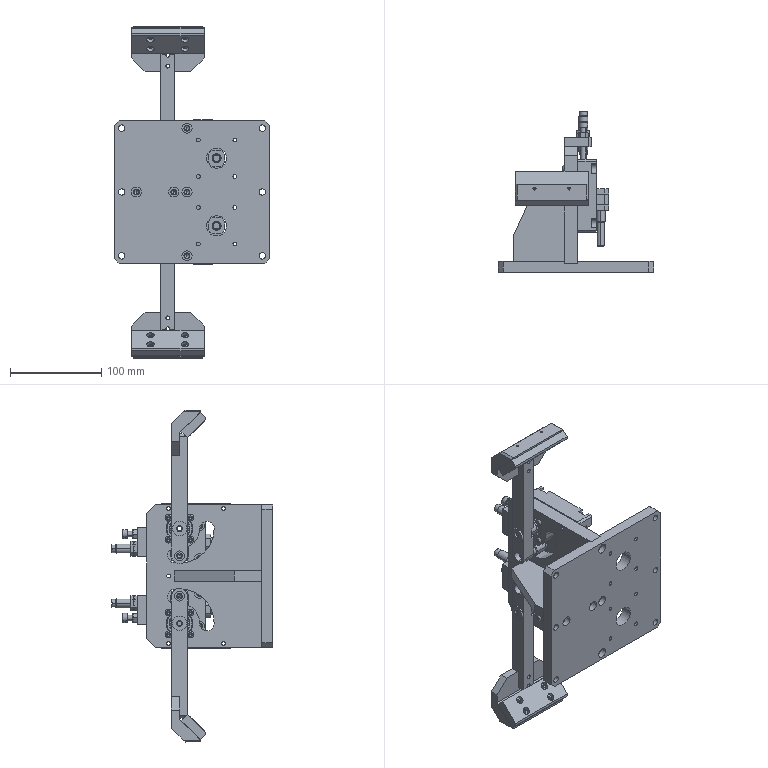Assembly | SolidWorks | mm | 57 component files | 57 solids | 1432 faces | box 170 x 176.7 x 364.01 mm | volume 992692 mm3 | plane 567 | cylinder 496 | spline 179 | cone 174 | torus 16 | commonest cylinder face diameters 10 x64 4.2 x48 4 x32 5 x28 5.5 x28 11 x26 16 x22 6.6 x22
Bill of materials:
A26 | 2 | S45C | Plate of constant thickness bent once into two flat legs at an obtuse angle. The shorter leg has angled (chamfered) corners and two round holes; the longer rectangular leg has four smaller holes in a 2x2 pattern.
A27 | 2 | Urethane | Rectangular flat bar or plate with four counterbored holes in a 2x2 pattern; one end face appears to be cut at an angle.
A73 | 4 | S45C | Thin flat ring (annular disc) with a centered round through hole, like a plain washer.
A74 | 2 | S45C | Stepped round pin with three coaxial diameters: a large head with a chamfered end, a middle shank, and a smaller end shank with a small axial hole.
A75 | 2 | Brass | Plain cylindrical sleeve or bushing with a large through bore and chamfered outer edges at both ends.
A78 | 2 | S45C | Thin flat ring (annular disc) with a centered round through hole, like a plain washer; the hole is a little smaller relative to the outside diameter than in the similar ring.
A79 | 2 | S45C | Thicker flat ring or spacer disc with a fairly small centered through hole.
A87 | 1 | S45C | Long flat bar or link with one rounded end. It has a hole near the rounded end, a larger hole partway along, a stepped or notched side profile, and a narrower tail section with two small holes and a chamfered tip.
BPS01-d6 | 2 | Standard Part | Short thick cylinder or roller-like ring with a centered through bore, rounded or chamfered outer edges, and a small edge break at the bore.
A70 | 1 | S136 | Thick rectangular plate with two clipped corners on one side. It has two mirrored curved arc slots, two large round holes, a row of small and medium holes across the middle, small holes near the edges, and holes drilled into one edge face.
A72 | 2 | S45C | Stepped cylindrical bushing with a through bore. It has a large central collar with a small extra step on one side, and two shaft ends of different diameters with chamfered ends.
A76 | 2 | S136 | Rectangular block or plate with two clipped corners on one side, a large obround (stadium-shaped) through slot, and two round holes in a stepped flange strip along the opposite side.
A77 | 2 | S45C | Thick, nearly square block or plate with two chamfered corners on one side and four through holes: three smaller holes and one larger hole.
A80 | 2 | S45C | Rectangular block with chamfered corners on one long side and a U-shaped slot with a rounded end cut through its full thickness, open on that side.
A81 | 2 | S45C | Stepped shaft or pin on one axis, with two spaced flanges that have chamfered corners, a middle shoulder diameter, and a long, smaller-diameter pin end.
A82 | 1 | S45C | Thin rectangular plate with small corner chamfers and a pattern of holes: two large through holes, several medium holes along the edges and center line, and small holes arranged in rows. A shallow notch is cut into one long edge.
A83 | 1 | A6061 | Flat block with a tapered planform: one end is narrowed by an angled cut. Drilled holes enter the long side faces.
A84 | 2 | S136 | Long rectangular bar with a raised step or tab region at one end of the profile, rounded-end notches cut into one side face, and two through holes along its length. The end corners are chamfered.
A85 | 1 | S136 | Long rectangular bar similar to a spacer or clamp bar, with two through holes near the ends, chamfered end corners, and a small stepped notch along one edge.
DeepGrooveBallBearing16001 | 2 | Standard Part | Annular rolling-element assembly: an outer ring, an inner ring and a single row of spherical balls between them. No cage or seals are visible. The geometry is consistent with a radial ball bearing.
M5X10 | 1 | Standard Part | Fastener-like part with a domed (button) head, a hexagonal socket recess and a plain cylindrical shank.
M6-N | 2 | Standard Part | Hexagonal nut-like part with a round central bore and chamfered corners on both faces.
M6X35-N | 2 | Standard Part | Headed cylindrical pin or simplified screw: a short cylindrical head of larger diameter with a long, plain, smaller-diameter shank.
PanHeadM4X8-N | 8 | Standard Part | Round-head, rivet- or pin-like part: a domed head with a flat underside and a plain cylindrical shank with a flat end.
RB1006-1 | 2 |  | Elongated, stepped cylindrical body. A long main barrel sits between a short, slightly narrower end section on one side and a short stepped collar on the other. A small solid cylindrical pin sticks out along the axis from the collar end. The opposite end section has a small notch or slot cut into its edge.
RB1006-2 | 2 |  | Thin hexagonal ring with a large plain central through-bore. The outer corners are chamfered on both faces, which leaves curved boundaries on the side flats. Its overall shape matches a thin hex nut.
RB1006-3 | 2 |  | Thin hexagonal ring with a large plain central through-bore. The outer corners are chamfered on both faces, which leaves curved boundaries on the side flats. Its overall shape matches a thin hex nut.
A89 | 1 | S45C | Long, narrow bar or plate with a roughly rectangular cross-section. One end is chamfered and squared off, and the other end is fully rounded. There are two small holes near the chamfered end and a larger hole partway down the bar. A side notch or pocket cuts in near the larger hole, and the rounded end has one more hole with an edge recess or counterbore. The bar steps in width near the chamfered end.
Mates:
1. coincident | ClampingAssembly-1/A72-1 face at (-35.551, 66.036, -52.5) dir (-1, 0, 0) | ClampingArm2-1/A87-1 face at (-35.551, 66.025, -85.5) dir (1, 0, 0)
2. parallel | ClampingAssembly-1/A72-1 face at (-37.551, 60.742, -58.498) dir (0, -0.0003333, -1) | ClampingArm2-1/A87-1 face at (-38.051, 75.034, -58.503) dir (0, 0.0003333, 1)
3. concentric | ClampingAssembly-1/A72-1 face at (-49.551, 66.036, -52.5) dir (1, 0, 0) r 5 | ClampingArm2-1/A87-1 face at (-50.551, 66.036, -52.5) dir (1, 0, 0) r 5
4. cam | ClampingAssembly-1/A76-1 face at (-14.551, 56.526, -21.5) dir (0, 1, 0) | ClampingArm2-1/BPS01-d6-1 face at (-2.651, 66.046, -22.5) dir (-1, 0, 0) r 9.5
5. coincident | ClampingArm2-1/A87-1 face at (-50.551, 66.025, -85.5) dir (-1, 0, 0) | Reverse-ClampingArm2-1/A89-1 face at (-50.551, 66.047, 84.5) dir (-1, 0, 0)
6. parallel | ClampingAssembly-1/A72-2 face at (-37.551, 71.329, 57.498) dir (0, 0.0003333, 1) | Reverse-ClampingArm2-1/A89-1 face at (-38.051, 57.038, 57.503) dir (0, -0.0003333, -1)
7. cam | ClampingAssembly-1/A76-3 face at (-14.551, 66.036, 20.5) dir (1, 0, 0) r 9.51 | Reverse-ClampingArm2-1/BPS01-d6-1 face at (-2.651, 66.026, 21.5) dir (-1, 0, 0) r 9.5
8. parallel | ClampingAssembly-1/A72-2 face at (-37.551, 60.742, 45.502) dir (0, -0.0003333, -1) | Reverse-ClampingArm2-1/A89-1 face at (-38.051, 57.034, 45.503) dir (0, 0.0003333, 1)
9. concentric | ClampingAssembly-1/A72-2 face at (-49.551, 66.036, 51.5) dir (1, 0, 0) r 5 | Reverse-ClampingArm2-1/A89-1 face at (-50.551, 66.036, 51.5) dir (1, 0, 0) r 5
10. coincident | A87-1 face at (-0.2508, 28.779, -71) dir (0, 1, 0) | A26-1 face at (47.249, 28.779, -47) dir (0, -1, 0)
11. concentric | A87-1 face at (7.249, 28.779, -53) dir (0, 1, 0) r 2.1 | A26-1 face at (7.249, 37.779, -53) dir (0, 1, 0) r 2.75
12. concentric | A87-1 face at (7.249, 28.779, -65) dir (0, 1, 0) r 2.1 | A26-1 face at (7.249, 37.779, -65) dir (0, 1, 0) r 2.75
13. coincident | A26-1 face at (47.249, 28.779, -72) dir (0, -0.7071, 0.7071) | A27-1 face at (7.249, 16.672, -84.107) dir (0, 0.7071, -0.7071)
14. concentric | A26-1 face at (-11.751, 21.622, -79.157) dir (0, -0.7071, 0.7071) r 1.65 | A27-1 face at (-11.751, 14.551, -72.086) dir (0, -0.7071, 0.7071) r 2.25
15. concentric | A26-1 face at (26.249, 21.622, -79.157) dir (0, -0.7071, 0.7071) r 1.65 | A27-1 face at (26.249, 14.551, -72.086) dir (0, -0.7071, 0.7071) r 2.25
16. coincident | A87-1 face at (-0.2508, 28.779, 0) dir (-1, 0, 0) | A73-1 face at (-0.2508, 28.779, 33) dir (1, 0, 0)
17. concentric | A87-1 face at (-0.2508, 28.779, 33) dir (1, 0, 0) r 5 | A73-1 face at (-0.2508, 28.779, 33) dir (-1, 0, 0) r 3.25
18. concentric | A87-1 face at (-0.2508, 28.779, 63) dir (1, 0, 0) r 3.25 | A74-1 face at (20.749, 28.779, 63) dir (-1, 0, 0) r 7
19. coincident | A87-1 face at (12.749, 28.779, 63) dir (1, 0, 0) | A74-1 face at (12.749, 28.779, 63) dir (-1, 0, 0)
20. concentric | A74-1 face at (35.749, 28.779, 63) dir (-1, 0, 0) r 5 | A75-1 face at (35.249, 28.779, 63) dir (-1, 0, 0) r 8
21. width | A75-1 face at (21.249, 28.779, 63) dir (-1, 0, 0) | A75-1 face at (35.249, 28.779, 63) dir (1, 0, 0) | A74-1 face at (20.749, 28.779, 63) dir (1, 0, 0) | A74-1 face at (35.749, 28.779, 63) dir (1, 0, 0)
22. concentric | A74-1 face at (47.749, 28.779, 63) dir (-1, 0, 0) r 3 | A78-1 face at (37.749, 28.779, 63) dir (-1, 0, 0) r 3.1
23. coincident | A74-1 face at (35.749, 28.779, 63) dir (1, 0, 0) | A78-1 face at (35.749, 28.779, 63) dir (-1, 0, 0)
24. concentric | A74-1 face at (47.749, 28.779, 63) dir (-1, 0, 0) r 3 | BPS01-d6-1 face at (47.649, 28.779, 63) dir (-1, 0, 0) r 9.5
25. coincident | A78-1 face at (37.749, 28.779, 63) dir (1, 0, 0) | BPS01-d6-1 face at (37.749, 28.779, 63) dir (-1, 0, 0)
26. coincident | A74-1 face at (47.749, 28.779, 63) dir (1, 0, 0) | A79-1 face at (47.749, 28.779, 63) dir (-1, 0, 0)
27. concentric | A74-1 face at (47.749, 28.779, 63) dir (1, 0, 0) r 1.25 | A79-1 face at (49.749, 28.779, 63) dir (-1, 0, 0) r 5
28. parallel | A87-1 face at (14.749, 37.779, 71) dir (0, 1, 0) | A73-1 plane at (-1.251, 28.779, 33) dir (0, 1, 0)
29. parallel | A87-1 face at (14.749, 37.779, 71) dir (0, 1, 0) | A74-1 plane at (16.749, 28.779, 63) dir (0, -1, 0)
30. parallel | A87-1 face at (14.749, 37.779, 71) dir (0, 1, 0) | A75-1 plane at (28.249, 28.779, 63) dir (0, -1, 0)
31. parallel | A87-1 face at (14.749, 37.779, 71) dir (0, 1, 0) | A78-1 plane at (35.749, 28.779, 63) dir (0, 1, 0)
32. parallel | A87-1 face at (14.749, 37.779, 71) dir (0, 1, 0) | BPS01-d6-1 plane at (42.749, 28.779, 63) dir (0, -1, 0)
33. parallel | A87-1 face at (14.749, 37.779, 71) dir (0, 1, 0) | A79-1 plane at (48.749, 28.779, 63) dir (0, 1, 0)
34. concentric | A70-1 face at (7.478, 54.35, -52) dir (-1, 0, 0) r 14 | DeepGrooveBallBearing16001-1 face at (-4.733, 54.35, -52) dir (-1, 0, 0) r 14
35. coincident | A70-1 face at (7.478, 54.35, -52) dir (-1, 0, 0) | DeepGrooveBallBearing16001-1 face at (7.478, 68.35, -52) dir (1, 0, 0)
36. parallel | A70-1 face at (15.478, 90.35, -78) dir (0, 0, -1) | DeepGrooveBallBearing16001-1 plane at (3.978, 54.35, -52) dir (0, 0, 1)
37. concentric | DeepGrooveBallBearing16001-1 face at (-2.994, 54.35, -52) dir (-1, 0, 0) r 6 | A72-1 face at (7.478, 54.35, -52) dir (-1, 0, 0) r 6
38. coincident | DeepGrooveBallBearing16001-1 face at (0.4778, 63.017, -52) dir (-1, 0, 0) | A72-1 face at (0.4778, 54.35, -52) dir (1, 0, 0)
39. concentric | A70-1 face at (0.4778, 66.371, -64.021) dir (-1, 0, 0) r 2 | PanHeadM4X8-N-1 face at (8.478, 66.371, -64.021) dir (-1, 0, 0) r 2
40. coincident | A70-1 face at (0.4778, 26.35, 0) dir (-1, 0, 0) | PanHeadM4X8-N-1 face at (0.4778, 66.371, -64.021) dir (1, 0, 0)
41. parallel | A70-1 face at (15.478, 90.35, -78) dir (0, 0, -1) | PanHeadM4X8-N-1 face at (-0.4222, 67.093, -62.771) dir (0, 0, -1)
42. concentric | A70-1 face at (0.4778, 42.329, -64.021) dir (-1, 0, 0) r 2 | PanHeadM4X8-N-2 face at (8.478, 42.329, -64.021) dir (-1, 0, 0) r 2
43. coincident | A70-1 face at (0.4778, 26.35, 0) dir (-1, 0, 0) | PanHeadM4X8-N-2 face at (0.4778, 42.329, -64.021) dir (1, 0, 0)
44. parallel | A70-1 face at (15.478, 90.35, -78) dir (0, 0, -1) | PanHeadM4X8-N-2 face at (-0.4222, 43.051, -62.771) dir (0, 0, -1)
45. concentric | A70-1 face at (0.4778, 42.329, -39.979) dir (-1, 0, 0) r 2 | PanHeadM4X8-N-4 face at (8.478, 42.329, -39.979) dir (-1, 0, 0) r 2
46. coincident | A70-1 face at (0.4778, 26.35, 0) dir (-1, 0, 0) | PanHeadM4X8-N-4 face at (0.4778, 42.329, -39.979) dir (1, 0, 0)
47. parallel | A70-1 face at (15.478, 90.35, -78) dir (0, 0, -1) | PanHeadM4X8-N-4 face at (-0.4222, 43.051, -38.729) dir (0, 0, -1)
48. concentric | A70-1 face at (0.4778, 66.371, -39.979) dir (-1, 0, 0) r 2 | PanHeadM4X8-N-6 face at (8.478, 66.371, -39.979) dir (-1, 0, 0) r 2
49. coincident | A70-1 face at (0.4778, 26.35, 0) dir (-1, 0, 0) | PanHeadM4X8-N-6 face at (0.4778, 66.371, -39.979) dir (1, 0, 0)
50. parallel | A70-1 face at (15.478, 90.35, -78) dir (0, 0, -1) | PanHeadM4X8-N-6 face at (-0.4222, 67.093, -38.729) dir (0, 0, -1)
51. coincident | A72-1 face at (7.478, 54.35, -52) dir (1, 0, 0) | A73-1 face at (7.478, 54.35, -52) dir (-1, 0, 0)
52. concentric | A72-1 face at (7.478, 54.35, -52) dir (1, 0, 0) r 2.5 | A73-1 face at (9.478, 54.35, -52) dir (-1, 0, 0) r 3.25
53. coincident | A70-1 face at (15.478, 26.35, 0) dir (1, 0, 0) | A76-1 face at (15.478, 51.35, -37) dir (-1, 0, 0)
54. coincident | A73-1 face at (9.478, 54.35, -52) dir (1, 0, 0) | M5X10-1 face at (9.478, 54.35, -52) dir (-1, 0, 0)
55. concentric | A72-1 face at (7.478, 54.35, -52) dir (1, 0, 0) r 2.5 | M5X10-1 face at (-0.5222, 54.35, -52) dir (1, 0, 0) r 2.5
56. distance | DeepGrooveBallBearing16001-1 plane at (3.978, 54.35, -52) dir (0, 0, 1) | A76-1 face at (27.478, 76.35, -5) dir (0, 0, 1)
57. coincident | A70-1 face at (15.478, 90.35, 78) dir (0, 1, 0) | A77-1 face at (15.478, 90.35, -37) dir (0, -1, 0)
58. coincident | A70-1 face at (0.4778, 26.35, 0) dir (-1, 0, 0) | A77-1 face at (0.4778, 100.35, -53) dir (-1, 0, 0)
59. width | A77-1 face at (30.478, 100.35, -21) dir (0, 0, 1) | A77-1 face at (30.478, 100.35, -53) dir (0, 0, -1) | A76-1 face at (27.478, 76.35, -69) dir (0, 0, -1) | A76-1 face at (27.478, 76.35, -5) dir (0, 0, 1)
60. concentric | A77-1 face at (21.478, 100.35, -30) dir (0, 1, 0) r 5 | RB1006-1/RB1006-1-1 face at (21.478, 104.55, -30) dir (0, 1, 0) r 5
61. coincident | A77-1 face at (15.478, 100.35, -37) dir (0, 1, 0) | RB1006-1/RB1006-3-1 face at (21.478, 100.35, -36) dir (0, -1, 0)
62. parallel | A77-1 face at (30.478, 100.35, -53) dir (1, 0, 0) | RB1006-1/RB1006-3-1 face at (28.478, 104.35, -34.041) dir (1, 0, 0)
63. concentric | A77-1 face at (21.478, 100.35, -46) dir (0, 1, 0) r 3 | M6X35-N-1 face at (21.478, 76.35, -46) dir (0, 1, 0) r 3
64. coincident | RB1006-1/RB1006-1-1 face at (21.478, 76.35, -30) dir (0, -1, 0) | M6X35-N-1 face at (21.478, 76.35, -46) dir (0, -1, 0)
65. parallel | A77-1 face at (30.478, 100.35, -53) dir (1, 0, 0) | M6X35-N-1 face at (18.978, 114.35, -44.557) dir (1, 0, 0)
66. coincident | A77-1 face at (15.478, 100.35, -37) dir (0, 1, 0) | M6-N-1 face at (12.818, 100.35, -41) dir (0, -1, 0)
67. parallel | A77-1 face at (30.478, 100.35, -53) dir (0, 0, -1) | M6-N-1 face at (18.591, 105.55, -51) dir (0, 0, -1)
68. coincident | A76-1 face at (25.478, 51.35, -37) dir (1, 0, 0) | A80-1 face at (25.478, 38.35, -61) dir (-1, 0, 0)
69. coincident | A76-1 face at (27.478, 26.35, -5) dir (0, -1, 0) | A80-1 face at (37.478, 26.35, -37) dir (0, -1, 0)
70. width | A80-1 face at (49.478, 38.35, -13) dir (0, 0, 1) | A80-1 face at (49.478, 38.35, -61) dir (0, 0, -1) | A76-1 face at (27.478, 76.35, -69) dir (0, 0, -1) | A76-1 face at (27.478, 76.35, -5) dir (0, 0, 1)
71. coincident | A80-1 face at (37.478, 38.35, -37) dir (0, 1, 0) | A81-1 face at (40.478, 38.35, -37) dir (0, -1, 0)
72. width | A81-1 face at (49.478, 20.35, -46) dir (0, 0, -1) | A81-1 face at (49.478, 20.35, -28) dir (0, 0, 1) | A80-1 face at (49.478, 38.35, -13) dir (0, 0, 1) | A80-1 face at (49.478, 38.35, -61) dir (0, 0, -1)
73. distance | A81-1 plane at (40.478, 32.35, -37) dir (1, 0, 0) | A80-1 face at (49.478, 38.35, -61) dir (1, 0, 0)
74. distance | A82-1 face at (13.478, -35.65, 0) dir (0, 1, 0) | A70-1 face at (15.478, -37.65, 78) dir (0, -1, 0)
75. distance | A82-1 face at (98.478, -35.65, -78) dir (1, 0, 0) | A70-1 face at (15.478, 26.35, 0) dir (1, 0, 0)
76. coincident | A82-1 face at (13.478, -35.65, 0) dir (0, 1, 0) | A83-1 face at (-54.522, -35.65, 6) dir (0, -1, 0)
77. coincident | A70-1 face at (0.4778, 26.35, 0) dir (-1, 0, 0) | A83-1 face at (0.4778, -35.65, 6) dir (1, 0, 0)
78. coincident | A70-1 face at (15.478, 26.35, 0) dir (1, 0, 0) | A85-1 face at (15.478, 36.35, -2.5) dir (-1, 0, 0)
79. distance | A85-1 face at (35.478, 76.35, 5) dir (0, 1, 0) | A70-1 face at (15.478, 90.35, 78) dir (0, 1, 0)
80. coincident | A85-1 face at (35.478, 76.35, 5) dir (0, 1, 0) | A84-2 face at (35.478, 76.35, -79) dir (0, 1, 0)
81. coincident | A70-1 face at (15.478, 26.35, 0) dir (1, 0, 0) | A84-2 face at (15.478, 36.35, -71.5) dir (-1, 0, 0)
82. coincident | A70-1 face at (15.478, 90.35, -78) dir (0, 0, -1) | A82-1 face at (-71.522, -35.65, -78) dir (0, 0, -1)
83. coincident | A76-1 face at (27.478, 76.35, -5) dir (0, 0, 1) | A85-1 face at (15.478, -3.65, -5) dir (0, 0, -1)
84. coincident | A70-1 face at (7.478, 54.35, 52) dir (-1, 0, 0) | DeepGrooveBallBearing16001-2 face at (7.478, 68.35, 52) dir (1, 0, 0)
85. concentric | A70-1 face at (7.478, 54.35, 52) dir (-1, 0, 0) r 14 | DeepGrooveBallBearing16001-2 face at (-4.733, 54.35, 52) dir (-1, 0, 0) r 14
86. parallel | A70-1 face at (15.478, 90.35, 78) dir (0, 0, 1) | DeepGrooveBallBearing16001-2 plane at (3.978, 54.35, 52) dir (0, 0, 1)
87. concentric | DeepGrooveBallBearing16001-2 face at (-2.994, 54.35, 52) dir (-1, 0, 0) r 6 | A72-2 face at (7.478, 54.35, 52) dir (-1, 0, 0) r 6
88. coincident | DeepGrooveBallBearing16001-2 face at (0.4778, 63.017, 52) dir (-1, 0, 0) | A72-2 face at (0.4778, 54.35, 52) dir (1, 0, 0)
89. coincident | A72-2 face at (7.478, 54.35, 52) dir (1, 0, 0) | A73-6 face at (7.478, 54.35, 52) dir (-1, 0, 0)
90. concentric | A72-2 face at (7.478, 54.35, 52) dir (1, 0, 0) r 2.5 | A73-6 face at (9.478, 54.35, 52) dir (-1, 0, 0) r 3.25
91. coincident | A84-2 face at (35.478, 76.35, -79) dir (0, 1, 0) | A84-3 face at (35.557, 76.35, 79) dir (0, 1, 0)
92. coincident | A70-1 face at (15.478, 26.35, 0) dir (1, 0, 0) | A76-3 face at (15.478, 51.35, 37) dir (-1, 0, 0)
93. coincident | A76-1 face at (27.478, 76.35, -5) dir (0, 1, 0) | A76-3 face at (27.478, 76.35, 69) dir (0, 1, 0)
94. distance | DeepGrooveBallBearing16001-2 plane at (3.978, 54.35, 52) dir (0, 0, 1) | A76-3 face at (27.478, 76.35, 5) dir (0, 0, -1)
95. coincident | A70-1 face at (15.478, 90.35, 78) dir (0, 1, 0) | A77-3 face at (15.478, 90.35, 37) dir (0, -1, 0)
96. coincident | A70-1 face at (0.4778, 26.35, 0) dir (-1, 0, 0) | A77-3 face at (0.4778, 90.35, 53) dir (-1, 0, 0)
97. width | A77-3 face at (30.478, 90.35, 53) dir (0, 0, 1) | A77-3 face at (30.478, 90.35, 21) dir (0, 0, -1) | A84-3 face at (15.557, -3.65, 69) dir (0, 0, -1) | A85-1 face at (35.478, -3.65, 5) dir (0, 0, 1)
98. coincident | A84-3 face at (15.557, -3.65, 69) dir (0, 0, -1) | A76-3 face at (27.478, 76.35, 69) dir (0, 0, 1)
99. coincident | A76-3 face at (25.478, 51.35, 37) dir (1, 0, 0) | A80-2 face at (25.478, 38.35, 13) dir (-1, 0, 0)
100. coincident | A76-3 face at (25.478, 38.35, 69) dir (0, -1, 0) | A80-2 face at (37.478, 38.35, 37) dir (0, 1, 0)
101. width | A80-2 face at (49.478, 38.35, 61) dir (0, 0, 1) | A80-2 face at (49.478, 38.35, 13) dir (0, 0, -1) | A84-3 face at (15.557, -3.65, 69) dir (0, 0, -1) | A85-1 face at (35.478, -3.65, 5) dir (0, 0, 1)
102. concentric | A77-3 face at (21.478, 90.35, 30) dir (0, -1, 0) r 5 | RB1006-2/RB1006-1-1 face at (21.478, 104.55, 30) dir (0, 1, 0) r 5
103. coincident | A77-3 face at (15.478, 100.35, 37) dir (0, 1, 0) | RB1006-2/RB1006-3-1 face at (21.478, 100.35, 24) dir (0, -1, 0)
104. parallel | A77-3 face at (30.478, 90.35, 53) dir (1, 0, 0) | RB1006-2/RB1006-3-1 face at (28.478, 104.35, 25.959) dir (1, 0, 0)
105. concentric | A77-3 face at (21.478, 90.35, 46) dir (0, -1, 0) r 3 | M6X35-N-2 face at (21.478, 76.35, 46) dir (0, 1, 0) r 3
106. coincident | RB1006-2/RB1006-1-1 face at (21.478, 76.35, 30) dir (0, -1, 0) | M6X35-N-2 face at (21.478, 76.35, 46) dir (0, -1, 0)
107. parallel | A77-3 face at (30.478, 90.35, 53) dir (1, 0, 0) | M6X35-N-2 face at (18.978, 114.35, 47.443) dir (1, 0, 0)
108. coincident | A77-3 face at (15.478, 100.35, 37) dir (0, 1, 0) | M6-N-2 face at (12.818, 100.35, 51) dir (0, -1, 0)
109. parallel | A77-3 face at (30.478, 90.35, 53) dir (0, 0, 1) | M6-N-2 face at (24.365, 105.55, 51) dir (0, 0, 1)
110. width | A81-2 face at (49.478, 20.35, 28) dir (0, 0, -1) | A81-2 face at (49.478, 20.35, 46) dir (0, 0, 1) | A80-2 face at (49.478, 38.35, 30.7) dir (0, 0, 1) | A80-2 face at (49.478, 38.35, 43.3) dir (0, 0, -1)
111. coincident | A80-2 face at (37.478, 38.35, 37) dir (0, 1, 0) | A81-2 face at (40.478, 38.35, 37) dir (0, -1, 0)
112. coincident | A81-1 face at (49.478, 20.35, -46) dir (1, 0, 0) | A81-2 face at (49.478, 20.35, 28) dir (1, 0, 0)
113. concentric | A70-1 face at (0.4778, 42.329, 39.979) dir (-1, 0, 0) r 2 | PanHeadM4X8-N-7 face at (8.478, 42.329, 39.979) dir (-1, 0, 0) r 2
114. coincident | A70-1 face at (0.4778, 26.35, 0) dir (-1, 0, 0) | PanHeadM4X8-N-7 face at (0.4778, 42.329, 39.979) dir (1, 0, 0)
115. parallel | A70-1 face at (15.478, 90.35, -78) dir (0, 0, -1) | PanHeadM4X8-N-7 face at (-0.4222, 43.051, 41.229) dir (0, 0, -1)
116. concentric | A70-1 face at (0.4778, 42.329, 64.021) dir (-1, 0, 0) r 2 | PanHeadM4X8-N-9 face at (8.478, 42.329, 64.021) dir (-1, 0, 0) r 2
117. coincident | A70-1 face at (0.4778, 26.35, 0) dir (-1, 0, 0) | PanHeadM4X8-N-9 face at (0.4778, 42.329, 64.021) dir (1, 0, 0)
118. parallel | A70-1 face at (15.478, 90.35, -78) dir (0, 0, -1) | PanHeadM4X8-N-9 face at (-0.4222, 43.051, 65.271) dir (0, 0, -1)
119. concentric | A70-1 face at (0.4778, 66.371, 64.021) dir (-1, 0, 0) r 2 | PanHeadM4X8-N-11 face at (8.478, 66.371, 64.021) dir (-1, 0, 0) r 2
120. coincident | A70-1 face at (0.4778, 26.35, 0) dir (-1, 0, 0) | PanHeadM4X8-N-11 face at (0.4778, 66.371, 64.021) dir (1, 0, 0)
121. parallel | A70-1 face at (15.478, 90.35, -78) dir (0, 0, -1) | PanHeadM4X8-N-11 face at (-0.4222, 67.093, 65.271) dir (0, 0, -1)
122. concentric | A70-1 face at (0.4778, 66.371, 39.979) dir (-1, 0, 0) r 2 | PanHeadM4X8-N-14 face at (8.478, 66.371, 39.979) dir (-1, 0, 0) r 2
123. coincident | A70-1 face at (0.4778, 26.35, 0) dir (-1, 0, 0) | PanHeadM4X8-N-14 face at (0.4778, 66.371, 39.979) dir (1, 0, 0)
124. parallel | A70-1 face at (15.478, 90.35, -78) dir (0, 0, -1) | PanHeadM4X8-N-14 face at (-0.4222, 67.093, 41.229) dir (0, 0, -1)
125. width | A83-1 face at (-27.022, 12.35, -6) dir (0, 0, -1) | A83-1 face at (-27.022, 12.35, 6) dir (0, 0, 1) | A70-1 face at (15.478, 90.35, -78) dir (0, 0, -1) | A70-1 face at (15.478, 90.35, 78) dir (0, 0, 1)
126. distance | A76-1 face at (27.478, 76.35, -5) dir (0, 1, 0) | A70-1 face at (15.478, 90.35, 78) dir (0, 1, 0)
127. coincident | A76-1 face at (27.478, 76.35, -69) dir (0, 0, -1) | A84-2 face at (15.478, 76.35, -69) dir (0, 0, 1)
128. concentric | M6X35-N-1 face at (21.478, 76.35, -46) dir (0, 1, 0) r 3 | M6-N-1 face at (21.478, 105.55, -46) dir (0, -1, 0) r 3
129. concentric | M6X35-N-2 face at (21.478, 76.35, 46) dir (0, 1, 0) r 3 | M6-N-2 face at (21.478, 105.55, 46) dir (0, -1, 0) r 3
130. distance | RB1006-3-1 face at (18, -6, 0) dir (-1, 0, 0) | RB1006-1-1 face at (-6, 0, 0) dir (-1, 0, 0)
131. coincident | RB1006-2-1 face at (22, 6, 0) dir (-1, 0, 0) | RB1006-3-1 face at (22, -6, 0) dir (1, 0, 0)
132. coincident | RB1006-2-1 face at (22, 8.083, 0) dir (0, 0.866, 0.5) | RB1006-3-1 face at (22, 4.041, 7) dir (0, 0.866, 0.5)
133. concentric | RB1006-1-1 face at (22.2, 0, 0) dir (1, 0, 0) r 5 | RB1006-3-1 face at (18, 0, 0) dir (-1, 0, 0) r 5
134. concentric | RB1006-1-1 face at (22.2, 0, 0) dir (1, 0, 0) r 5 | RB1006-2-1 face at (22, 0, 0) dir (-1, 0, 0) r 5
135. coincident | A89-1 face at (-9.722, 19.064, -71) dir (0, -1, 0) | A26-1 face at (-42.222, 19.064, -47) dir (0, 1, 0)
136. concentric | A89-1 face at (-2.222, 19.064, -65) dir (0, -1, 0) r 2.1 | A26-1 face at (-2.222, 10.064, -65) dir (0, -1, 0) r 5
137. concentric | A89-1 face at (-2.222, 19.064, -53) dir (0, -1, 0) r 2.1 | A26-1 face at (-2.222, 10.064, -53) dir (0, -1, 0) r 2.75
138. coincident | A26-1 face at (-42.222, 19.064, -72) dir (0, 0.7071, 0.7071) | A27-1 face at (-2.222, 31.171, -84.107) dir (0, -0.7071, -0.7071)
139. concentric | A26-1 face at (16.778, 36.121, -89.056) dir (0, 0.7071, 0.7071) r 1.65 | A27-1 face at (16.778, 43.192, -81.985) dir (0, 0.7071, 0.7071) r 2.25
140. concentric | A26-1 face at (-21.222, 26.221, -79.157) dir (0, 0.7071, 0.7071) r 1.65 | A27-1 face at (-21.222, 33.292, -72.086) dir (0, 0.7071, 0.7071) r 2.25
141. coincident | A89-1 face at (-9.722, 19.064, 0) dir (-1, 0, 0) | A73-1 face at (-9.722, 19.064, 33) dir (1, 0, 0)
142. concentric | A89-1 face at (-9.722, 19.064, 33) dir (1, 0, 0) r 5 | A73-1 face at (-9.722, 19.064, 33) dir (-1, 0, 0) r 3.25
143. concentric | A89-1 face at (-9.722, 19.064, 63) dir (1, 0, 0) r 3.25 | A74-1 face at (11.278, 19.064, 63) dir (-1, 0, 0) r 7
144. coincident | A89-1 face at (3.278, 19.064, 63) dir (1, 0, 0) | A74-1 face at (3.278, 19.064, 63) dir (-1, 0, 0)
145. concentric | A74-1 face at (26.278, 19.064, 63) dir (-1, 0, 0) r 5 | A75-1 face at (25.778, 19.064, 63) dir (-1, 0, 0) r 8
146. width | A75-1 face at (25.778, 19.064, 63) dir (1, 0, 0) | A75-1 face at (11.778, 19.064, 63) dir (-1, 0, 0) | A74-1 face at (11.278, 19.064, 63) dir (1, 0, 0) | A74-1 face at (26.278, 19.064, 63) dir (1, 0, 0)
147. concentric | A74-1 face at (38.278, 19.064, 63) dir (-1, 0, 0) r 3 | A78-1 face at (28.278, 19.064, 63) dir (-1, 0, 0) r 7
148. coincident | A74-1 face at (26.278, 19.064, 63) dir (1, 0, 0) | A78-1 face at (26.278, 19.064, 63) dir (-1, 0, 0)
149. concentric | A74-1 face at (38.278, 19.064, 63) dir (-1, 0, 0) r 3 | BPS01-d6-1 face at (38.178, 19.064, 63) dir (-1, 0, 0) r 9.5
150. coincident | A78-1 face at (28.278, 19.064, 63) dir (1, 0, 0) | BPS01-d6-1 face at (28.278, 19.064, 63) dir (-1, 0, 0)
151. concentric | A74-1 face at (38.278, 19.064, 63) dir (1, 0, 0) r 1.25 | A79-1 face at (40.278, 19.064, 63) dir (-1, 0, 0) r 1.75
152. coincident | A74-1 face at (38.278, 19.064, 63) dir (1, 0, 0) | A79-1 face at (38.278, 19.064, 63) dir (-1, 0, 0)
153. parallel | A89-1 face at (5.278, 28.064, 71) dir (0, 1, 0) | A73-1 plane at (-10.722, 19.064, 33) dir (0, -1, 0)
154. parallel | A89-1 face at (5.278, 28.064, 71) dir (0, 1, 0) | A74-1 plane at (7.278, 19.064, 63) dir (0, -1, 0)
155. parallel | A89-1 face at (5.278, 28.064, 71) dir (0, 1, 0) | A75-1 plane at (18.778, 19.064, 63) dir (0, -1, 0)
156. parallel | A89-1 face at (5.278, 28.064, 71) dir (0, 1, 0) | A78-1 plane at (26.278, 19.064, 63) dir (0, -1, 0)
157. parallel | A89-1 face at (5.278, 28.064, 71) dir (0, 1, 0) | BPS01-d6-1 plane at (33.278, 19.064, 63) dir (0, -1, 0)
158. parallel | A89-1 face at (5.278, 28.064, 71) dir (0, 1, 0) | A79-1 plane at (39.278, 19.064, 63) dir (0, -1, 0)